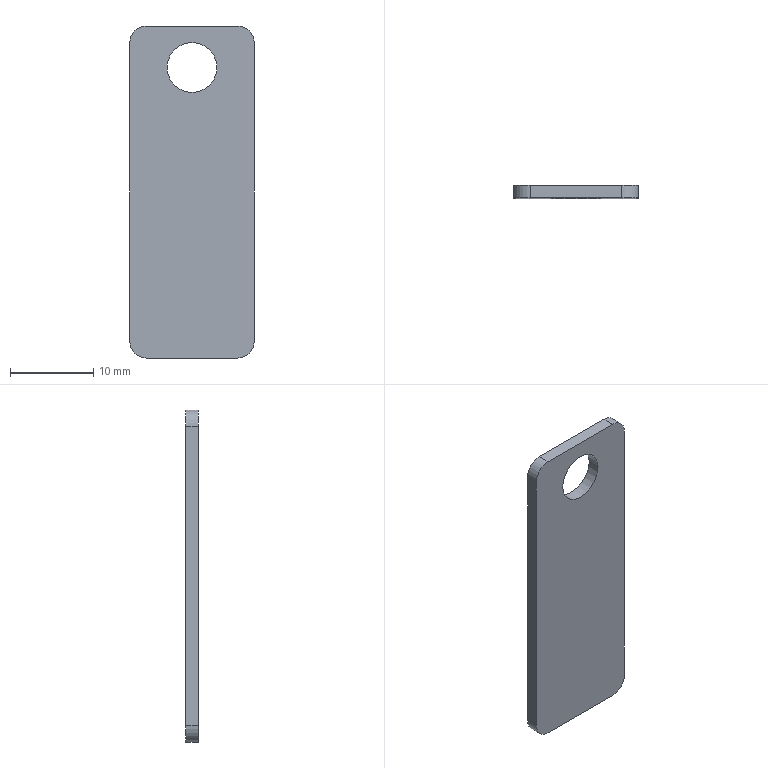Component | SolidWorks | FiberOpticBracket-1 | 1 solid | 12 faces | box 15 x 1.5 x 40 mm | volume 852 mm3 | cylinder 6 | plane 6 | commonest cylinder face diameters 4 x4 6 x2
STEP:
#1=COLOUR_RGB('',0.7922,0.8196,0.9333);
#2=FILL_AREA_STYLE_COLOUR('',#1);
#3=FILL_AREA_STYLE('',(#2));
#4=SURFACE_STYLE_FILL_AREA(#3);
#5=SURFACE_SIDE_STYLE('',(#4));
#6=SURFACE_STYLE_USAGE(.BOTH.,#5);
#7=PRESENTATION_STYLE_ASSIGNMENT((#6));
#8=CARTESIAN_POINT('',(-0.6049,-0.5041,4.668));
#9=VERTEX_POINT('',#8);
#10=CARTESIAN_POINT('',(-0.8411,-0.5041,4.668));
#11=VERTEX_POINT('',#10);
#12=CARTESIAN_POINT('',(-0.723,-0.5041,4.668));
#13=DIRECTION('',(-0.,1.,0.));
#14=DIRECTION('',(-1.,0.,0.));
#15=AXIS2_PLACEMENT_3D('',#12,#13,#14);
#16=CIRCLE('',#15,0.1181);
#17=EDGE_CURVE('',#9,#11,#16,.T.);
#18=ORIENTED_EDGE('',*,*,#17,.F.);
#19=CARTESIAN_POINT('',(-0.6049,-0.4451,4.668));
#20=VERTEX_POINT('',#19);
#21=CARTESIAN_POINT('',(-0.6049,-0.8388,4.668));
#22=DIRECTION('',(-0.,1.,0.));
#23=VECTOR('',#22,39.37);
#24=LINE('',#21,#23);
#25=EDGE_CURVE('',#9,#20,#24,.T.);
#26=ORIENTED_EDGE('',*,*,#25,.T.);
#27=CARTESIAN_POINT('',(-0.8411,-0.4451,4.668));
#28=VERTEX_POINT('',#27);
#29=CARTESIAN_POINT('',(-0.723,-0.4451,4.668));
#30=DIRECTION('',(-0.,1.,0.));
#31=DIRECTION('',(-1.,0.,0.));
#32=AXIS2_PLACEMENT_3D('',#29,#30,#31);
#33=CIRCLE('',#32,0.1181);
#34=EDGE_CURVE('',#20,#28,#33,.T.);
#35=ORIENTED_EDGE('',*,*,#34,.T.);
#36=CARTESIAN_POINT('',(-0.8411,-0.8388,4.668));
#37=DIRECTION('',(-0.,1.,0.));
#38=VECTOR('',#37,39.37);
#39=LINE('',#36,#38);
#40=EDGE_CURVE('',#11,#28,#39,.T.);
#41=ORIENTED_EDGE('',*,*,#40,.F.);
#42=EDGE_LOOP('',(#18,#26,#35,#41));
#43=FACE_OUTER_BOUND('',#42,.T.);
#44=CARTESIAN_POINT('',(-0.723,-0.8388,4.668));
#45=DIRECTION('',(-0.,1.,0.));
#46=DIRECTION('',(-1.,0.,0.));
#47=AXIS2_PLACEMENT_3D('',#44,#45,#46);
#48=CYLINDRICAL_SURFACE('',#47,0.1181);
#49=ADVANCED_FACE('',(#43),#48,.F.);
#50=CARTESIAN_POINT('',(-0.723,-0.5041,4.668));
#51=DIRECTION('',(-0.,1.,0.));
#52=DIRECTION('',(-1.,0.,0.));
#53=AXIS2_PLACEMENT_3D('',#50,#51,#52);
#54=CIRCLE('',#53,0.1181);
#55=EDGE_CURVE('',#11,#9,#54,.T.);
#56=ORIENTED_EDGE('',*,*,#55,.T.);
#57=ORIENTED_EDGE('',*,*,#17,.T.);
#58=EDGE_LOOP('',(#56,#57));
#59=FACE_BOUND('',#58,.T.);
#60=CARTESIAN_POINT('',(-0.4278,-0.5041,3.369));
#61=VERTEX_POINT('',#60);
#62=CARTESIAN_POINT('',(-0.4278,-0.5041,4.787));
#63=VERTEX_POINT('',#62);
#64=CARTESIAN_POINT('',(-0.4278,-0.5041,3.291));
#65=DIRECTION('',(-0.,-0.,1.));
#66=VECTOR('',#65,39.37);
#67=LINE('',#64,#66);
#68=EDGE_CURVE('',#61,#63,#67,.T.);
#69=ORIENTED_EDGE('',*,*,#68,.T.);
#70=CARTESIAN_POINT('',(-0.5065,-0.5041,4.865));
#71=VERTEX_POINT('',#70);
#72=CARTESIAN_POINT('',(-0.5065,-0.5041,4.787));
#73=DIRECTION('',(0.,-1.,0.));
#74=DIRECTION('',(-1.,0.,0.));
#75=AXIS2_PLACEMENT_3D('',#72,#73,#74);
#76=CIRCLE('',#75,0.07874);
#77=EDGE_CURVE('',#63,#71,#76,.T.);
#78=ORIENTED_EDGE('',*,*,#77,.T.);
#79=CARTESIAN_POINT('',(-0.9396,-0.5041,4.865));
#80=VERTEX_POINT('',#79);
#81=CARTESIAN_POINT('',(-1.018,-0.5041,4.865));
#82=DIRECTION('',(1.,0.,0.));
#83=VECTOR('',#82,39.37);
#84=LINE('',#81,#83);
#85=EDGE_CURVE('',#80,#71,#84,.T.);
#86=ORIENTED_EDGE('',*,*,#85,.F.);
#87=CARTESIAN_POINT('',(-1.018,-0.5041,4.787));
#88=VERTEX_POINT('',#87);
#89=CARTESIAN_POINT('',(-0.9396,-0.5041,4.787));
#90=DIRECTION('',(0.,-1.,0.));
#91=DIRECTION('',(-1.,0.,0.));
#92=AXIS2_PLACEMENT_3D('',#89,#90,#91);
#93=CIRCLE('',#92,0.07874);
#94=EDGE_CURVE('',#80,#88,#93,.T.);
#95=ORIENTED_EDGE('',*,*,#94,.T.);
#96=CARTESIAN_POINT('',(-1.018,-0.5041,3.369));
#97=VERTEX_POINT('',#96);
#98=CARTESIAN_POINT('',(-1.018,-0.5041,3.291));
#99=DIRECTION('',(-0.,-0.,1.));
#100=VECTOR('',#99,39.37);
#101=LINE('',#98,#100);
#102=EDGE_CURVE('',#97,#88,#101,.T.);
#103=ORIENTED_EDGE('',*,*,#102,.F.);
#104=CARTESIAN_POINT('',(-0.9396,-0.5041,3.291));
#105=VERTEX_POINT('',#104);
#106=CARTESIAN_POINT('',(-0.9396,-0.5041,3.369));
#107=DIRECTION('',(0.,-1.,0.));
#108=DIRECTION('',(-1.,0.,0.));
#109=AXIS2_PLACEMENT_3D('',#106,#107,#108);
#110=CIRCLE('',#109,0.07874);
#111=EDGE_CURVE('',#97,#105,#110,.T.);
#112=ORIENTED_EDGE('',*,*,#111,.T.);
#113=CARTESIAN_POINT('',(-0.5065,-0.5041,3.291));
#114=VERTEX_POINT('',#113);
#115=CARTESIAN_POINT('',(-1.018,-0.5041,3.291));
#116=DIRECTION('',(1.,0.,0.));
#117=VECTOR('',#116,39.37);
#118=LINE('',#115,#117);
#119=EDGE_CURVE('',#105,#114,#118,.T.);
#120=ORIENTED_EDGE('',*,*,#119,.T.);
#121=CARTESIAN_POINT('',(-0.5065,-0.5041,3.369));
#122=DIRECTION('',(0.,-1.,0.));
#123=DIRECTION('',(-1.,0.,0.));
#124=AXIS2_PLACEMENT_3D('',#121,#122,#123);
#125=CIRCLE('',#124,0.07874);
#126=EDGE_CURVE('',#114,#61,#125,.T.);
#127=ORIENTED_EDGE('',*,*,#126,.T.);
#128=EDGE_LOOP('',(#69,#78,#86,#95,#103,#112,#120,#127));
#129=FACE_OUTER_BOUND('',#128,.T.);
#130=CARTESIAN_POINT('',(-1.018,-0.5041,3.291));
#131=DIRECTION('',(-0.,1.,-0.));
#132=DIRECTION('',(-1.,-0.,-0.));
#133=AXIS2_PLACEMENT_3D('',#130,#131,#132);
#134=PLANE('',#133);
#135=ADVANCED_FACE('',(#59,#129),#134,.F.);
#136=ORIENTED_EDGE('',*,*,#85,.T.);
#137=CARTESIAN_POINT('',(-0.5065,-0.4451,4.865));
#138=VERTEX_POINT('',#137);
#139=CARTESIAN_POINT('',(-0.5065,-0.4451,4.865));
#140=DIRECTION('',(-0.,1.,0.));
#141=VECTOR('',#140,39.37);
#142=LINE('',#139,#141);
#143=EDGE_CURVE('',#71,#138,#142,.T.);
#144=ORIENTED_EDGE('',*,*,#143,.T.);
#145=CARTESIAN_POINT('',(-0.9396,-0.4451,4.865));
#146=VERTEX_POINT('',#145);
#147=CARTESIAN_POINT('',(-1.018,-0.4451,4.865));
#148=DIRECTION('',(1.,0.,0.));
#149=VECTOR('',#148,39.37);
#150=LINE('',#147,#149);
#151=EDGE_CURVE('',#146,#138,#150,.T.);
#152=ORIENTED_EDGE('',*,*,#151,.F.);
#153=CARTESIAN_POINT('',(-0.9396,-0.5041,4.865));
#154=DIRECTION('',(0.,-1.,0.));
#155=VECTOR('',#154,39.37);
#156=LINE('',#153,#155);
#157=EDGE_CURVE('',#146,#80,#156,.T.);
#158=ORIENTED_EDGE('',*,*,#157,.T.);
#159=EDGE_LOOP('',(#136,#144,#152,#158));
#160=FACE_OUTER_BOUND('',#159,.T.);
#161=CARTESIAN_POINT('',(-1.018,-0.4451,4.865));
#162=DIRECTION('',(-0.,-0.,1.));
#163=DIRECTION('',(1.,0.,0.));
#164=AXIS2_PLACEMENT_3D('',#161,#162,#163);
#165=PLANE('',#164);
#166=ADVANCED_FACE('',(#160),#165,.T.);
#167=CARTESIAN_POINT('',(-0.723,-0.4451,4.668));
#168=DIRECTION('',(-0.,1.,0.));
#169=DIRECTION('',(-1.,0.,0.));
#170=AXIS2_PLACEMENT_3D('',#167,#168,#169);
#171=CIRCLE('',#170,0.1181);
#172=EDGE_CURVE('',#28,#20,#171,.T.);
#173=ORIENTED_EDGE('',*,*,#172,.F.);
#174=ORIENTED_EDGE('',*,*,#34,.F.);
#175=EDGE_LOOP('',(#173,#174));
#176=FACE_BOUND('',#175,.T.);
#177=ORIENTED_EDGE('',*,*,#151,.T.);
#178=CARTESIAN_POINT('',(-0.4278,-0.4451,4.787));
#179=VERTEX_POINT('',#178);
#180=CARTESIAN_POINT('',(-0.5065,-0.4451,4.787));
#181=DIRECTION('',(-0.,1.,0.));
#182=DIRECTION('',(-1.,0.,0.));
#183=AXIS2_PLACEMENT_3D('',#180,#181,#182);
#184=CIRCLE('',#183,0.07874);
#185=EDGE_CURVE('',#138,#179,#184,.T.);
#186=ORIENTED_EDGE('',*,*,#185,.T.);
#187=CARTESIAN_POINT('',(-0.4278,-0.4451,3.369));
#188=VERTEX_POINT('',#187);
#189=CARTESIAN_POINT('',(-0.4278,-0.4451,3.291));
#190=DIRECTION('',(-0.,-0.,1.));
#191=VECTOR('',#190,39.37);
#192=LINE('',#189,#191);
#193=EDGE_CURVE('',#188,#179,#192,.T.);
#194=ORIENTED_EDGE('',*,*,#193,.F.);
#195=CARTESIAN_POINT('',(-0.5065,-0.4451,3.291));
#196=VERTEX_POINT('',#195);
#197=CARTESIAN_POINT('',(-0.5065,-0.4451,3.369));
#198=DIRECTION('',(-0.,1.,0.));
#199=DIRECTION('',(-1.,0.,0.));
#200=AXIS2_PLACEMENT_3D('',#197,#198,#199);
#201=CIRCLE('',#200,0.07874);
#202=EDGE_CURVE('',#188,#196,#201,.T.);
#203=ORIENTED_EDGE('',*,*,#202,.T.);
#204=CARTESIAN_POINT('',(-0.9396,-0.4451,3.291));
#205=VERTEX_POINT('',#204);
#206=CARTESIAN_POINT('',(-1.018,-0.4451,3.291));
#207=DIRECTION('',(1.,0.,0.));
#208=VECTOR('',#207,39.37);
#209=LINE('',#206,#208);
#210=EDGE_CURVE('',#205,#196,#209,.T.);
#211=ORIENTED_EDGE('',*,*,#210,.F.);
#212=CARTESIAN_POINT('',(-1.018,-0.4451,3.369));
#213=VERTEX_POINT('',#212);
#214=CARTESIAN_POINT('',(-0.9396,-0.4451,3.369));
#215=DIRECTION('',(-0.,1.,0.));
#216=DIRECTION('',(-1.,0.,0.));
#217=AXIS2_PLACEMENT_3D('',#214,#215,#216);
#218=CIRCLE('',#217,0.07874);
#219=EDGE_CURVE('',#205,#213,#218,.T.);
#220=ORIENTED_EDGE('',*,*,#219,.T.);
#221=CARTESIAN_POINT('',(-1.018,-0.4451,4.787));
#222=VERTEX_POINT('',#221);
#223=CARTESIAN_POINT('',(-1.018,-0.4451,3.291));
#224=DIRECTION('',(-0.,-0.,1.));
#225=VECTOR('',#224,39.37);
#226=LINE('',#223,#225);
#227=EDGE_CURVE('',#213,#222,#226,.T.);
#228=ORIENTED_EDGE('',*,*,#227,.T.);
#229=CARTESIAN_POINT('',(-0.9396,-0.4451,4.787));
#230=DIRECTION('',(-0.,1.,0.));
#231=DIRECTION('',(-1.,0.,0.));
#232=AXIS2_PLACEMENT_3D('',#229,#230,#231);
#233=CIRCLE('',#232,0.07874);
#234=EDGE_CURVE('',#222,#146,#233,.T.);
#235=ORIENTED_EDGE('',*,*,#234,.T.);
#236=EDGE_LOOP('',(#177,#186,#194,#203,#211,#220,#228,#235));
#237=FACE_OUTER_BOUND('',#236,.T.);
#238=CARTESIAN_POINT('',(-1.018,-0.4451,3.291));
#239=DIRECTION('',(-0.,1.,-0.));
#240=DIRECTION('',(-1.,-0.,-0.));
#241=AXIS2_PLACEMENT_3D('',#238,#239,#240);
#242=PLANE('',#241);
#243=ADVANCED_FACE('',(#176,#237),#242,.T.);
#244=ORIENTED_EDGE('',*,*,#210,.T.);
#245=CARTESIAN_POINT('',(-0.5065,-0.5041,3.291));
#246=DIRECTION('',(0.,-1.,0.));
#247=VECTOR('',#246,39.37);
#248=LINE('',#245,#247);
#249=EDGE_CURVE('',#196,#114,#248,.T.);
#250=ORIENTED_EDGE('',*,*,#249,.T.);
#251=ORIENTED_EDGE('',*,*,#119,.F.);
#252=CARTESIAN_POINT('',(-0.9396,-0.4451,3.291));
#253=DIRECTION('',(-0.,1.,0.));
#254=VECTOR('',#253,39.37);
#255=LINE('',#252,#254);
#256=EDGE_CURVE('',#105,#205,#255,.T.);
#257=ORIENTED_EDGE('',*,*,#256,.T.);
#258=EDGE_LOOP('',(#244,#250,#251,#257));
#259=FACE_OUTER_BOUND('',#258,.T.);
#260=CARTESIAN_POINT('',(-1.018,-0.5041,3.291));
#261=DIRECTION('',(0.,0.,-1.));
#262=DIRECTION('',(-1.,-0.,-0.));
#263=AXIS2_PLACEMENT_3D('',#260,#261,#262);
#264=PLANE('',#263);
#265=ADVANCED_FACE('',(#259),#264,.T.);
#266=ORIENTED_EDGE('',*,*,#102,.T.);
#267=CARTESIAN_POINT('',(-1.018,-0.4451,4.787));
#268=DIRECTION('',(-0.,1.,0.));
#269=VECTOR('',#268,39.37);
#270=LINE('',#267,#269);
#271=EDGE_CURVE('',#88,#222,#270,.T.);
#272=ORIENTED_EDGE('',*,*,#271,.T.);
#273=ORIENTED_EDGE('',*,*,#227,.F.);
#274=CARTESIAN_POINT('',(-1.018,-0.5041,3.369));
#275=DIRECTION('',(0.,-1.,0.));
#276=VECTOR('',#275,39.37);
#277=LINE('',#274,#276);
#278=EDGE_CURVE('',#213,#97,#277,.T.);
#279=ORIENTED_EDGE('',*,*,#278,.T.);
#280=EDGE_LOOP('',(#266,#272,#273,#279));
#281=FACE_OUTER_BOUND('',#280,.T.);
#282=CARTESIAN_POINT('',(-1.018,-0.4451,3.291));
#283=DIRECTION('',(1.,0.,0.));
#284=DIRECTION('',(0.,0.,-1.));
#285=AXIS2_PLACEMENT_3D('',#282,#283,#284);
#286=PLANE('',#285);
#287=ADVANCED_FACE('',(#281),#286,.F.);
#288=ORIENTED_EDGE('',*,*,#193,.T.);
#289=CARTESIAN_POINT('',(-0.4278,-0.4451,4.787));
#290=DIRECTION('',(0.,-1.,0.));
#291=VECTOR('',#290,39.37);
#292=LINE('',#289,#291);
#293=EDGE_CURVE('',#179,#63,#292,.T.);
#294=ORIENTED_EDGE('',*,*,#293,.T.);
#295=ORIENTED_EDGE('',*,*,#68,.F.);
#296=CARTESIAN_POINT('',(-0.4278,-0.4451,3.369));
#297=DIRECTION('',(-0.,1.,0.));
#298=VECTOR('',#297,39.37);
#299=LINE('',#296,#298);
#300=EDGE_CURVE('',#61,#188,#299,.T.);
#301=ORIENTED_EDGE('',*,*,#300,.T.);
#302=EDGE_LOOP('',(#288,#294,#295,#301));
#303=FACE_OUTER_BOUND('',#302,.T.);
#304=CARTESIAN_POINT('',(-0.4278,-0.4451,3.291));
#305=DIRECTION('',(1.,0.,0.));
#306=DIRECTION('',(0.,0.,-1.));
#307=AXIS2_PLACEMENT_3D('',#304,#305,#306);
#308=PLANE('',#307);
#309=ADVANCED_FACE('',(#303),#308,.T.);
#310=ORIENTED_EDGE('',*,*,#185,.F.);
#311=ORIENTED_EDGE('',*,*,#143,.F.);
#312=ORIENTED_EDGE('',*,*,#77,.F.);
#313=ORIENTED_EDGE('',*,*,#293,.F.);
#314=EDGE_LOOP('',(#310,#311,#312,#313));
#315=FACE_OUTER_BOUND('',#314,.T.);
#316=CARTESIAN_POINT('',(-0.5065,-0.4451,4.787));
#317=DIRECTION('',(0.,-1.,0.));
#318=DIRECTION('',(1.,0.,0.));
#319=AXIS2_PLACEMENT_3D('',#316,#317,#318);
#320=CYLINDRICAL_SURFACE('',#319,0.07874);
#321=ADVANCED_FACE('',(#315),#320,.T.);
#322=ORIENTED_EDGE('',*,*,#234,.F.);
#323=ORIENTED_EDGE('',*,*,#271,.F.);
#324=ORIENTED_EDGE('',*,*,#94,.F.);
#325=ORIENTED_EDGE('',*,*,#157,.F.);
#326=EDGE_LOOP('',(#322,#323,#324,#325));
#327=FACE_OUTER_BOUND('',#326,.T.);
#328=CARTESIAN_POINT('',(-0.9396,-0.4451,4.787));
#329=DIRECTION('',(-0.,1.,0.));
#330=DIRECTION('',(-1.,0.,0.));
#331=AXIS2_PLACEMENT_3D('',#328,#329,#330);
#332=CYLINDRICAL_SURFACE('',#331,0.07874);
#333=ADVANCED_FACE('',(#327),#332,.T.);
#334=ORIENTED_EDGE('',*,*,#126,.F.);
#335=ORIENTED_EDGE('',*,*,#249,.F.);
#336=ORIENTED_EDGE('',*,*,#202,.F.);
#337=ORIENTED_EDGE('',*,*,#300,.F.);
#338=EDGE_LOOP('',(#334,#335,#336,#337));
#339=FACE_OUTER_BOUND('',#338,.T.);
#340=CARTESIAN_POINT('',(-0.5065,-0.4451,3.369));
#341=DIRECTION('',(-0.,1.,0.));
#342=DIRECTION('',(-1.,0.,0.));
#343=AXIS2_PLACEMENT_3D('',#340,#341,#342);
#344=CYLINDRICAL_SURFACE('',#343,0.07874);
#345=ADVANCED_FACE('',(#339),#344,.T.);
#346=ORIENTED_EDGE('',*,*,#111,.F.);
#347=ORIENTED_EDGE('',*,*,#278,.F.);
#348=ORIENTED_EDGE('',*,*,#219,.F.);
#349=ORIENTED_EDGE('',*,*,#256,.F.);
#350=EDGE_LOOP('',(#346,#347,#348,#349));
#351=FACE_OUTER_BOUND('',#350,.T.);
#352=CARTESIAN_POINT('',(-0.9396,-0.5041,3.369));
#353=DIRECTION('',(0.,-1.,0.));
#354=DIRECTION('',(1.,0.,0.));
#355=AXIS2_PLACEMENT_3D('',#352,#353,#354);
#356=CYLINDRICAL_SURFACE('',#355,0.07874);
#357=ADVANCED_FACE('',(#351),#356,.T.);
#358=ORIENTED_EDGE('',*,*,#25,.F.);
#359=ORIENTED_EDGE('',*,*,#55,.F.);
#360=ORIENTED_EDGE('',*,*,#40,.T.);
#361=ORIENTED_EDGE('',*,*,#172,.T.);
#362=EDGE_LOOP('',(#358,#359,#360,#361));
#363=FACE_OUTER_BOUND('',#362,.T.);
#364=CARTESIAN_POINT('',(-0.723,-0.8388,4.668));
#365=DIRECTION('',(-0.,1.,0.));
#366=DIRECTION('',(-1.,0.,0.));
#367=AXIS2_PLACEMENT_3D('',#364,#365,#366);
#368=CYLINDRICAL_SURFACE('',#367,0.1181);
#369=ADVANCED_FACE('',(#363),#368,.F.);
#370=CLOSED_SHELL('',(#49,#135,#166,#243,#265,#287,#309,#321,#333,#345,#357,#369));
#371=MANIFOLD_SOLID_BREP('',#370);
#372=STYLED_ITEM('',(#7),#371);
#373=(LENGTH_UNIT()NAMED_UNIT(*)SI_UNIT($,.METRE.));
#374=LENGTH_MEASURE_WITH_UNIT(LENGTH_MEASURE(0.0254),#373);
#375=DIMENSIONAL_EXPONENTS(1.,0.,0.,0.,0.,0.,0.);
#376=(CONVERSION_BASED_UNIT('',#374)LENGTH_UNIT()NAMED_UNIT(#375));
#377=UNCERTAINTY_MEASURE_WITH_UNIT(LENGTH_MEASURE(0.00001),#376,'','');
#378=(NAMED_UNIT(*)PLANE_ANGLE_UNIT()SI_UNIT($,.RADIAN.));
#379=(NAMED_UNIT(*)SI_UNIT($,.STERADIAN.)SOLID_ANGLE_UNIT());
#380=(GEOMETRIC_REPRESENTATION_CONTEXT(3)GLOBAL_UNCERTAINTY_ASSIGNED_CONTEXT((#377))GLOBAL_UNIT_ASSIGNED_CONTEXT((#376,#378,#379))REPRESENTATION_CONTEXT('',''));
#381=MECHANICAL_DESIGN_GEOMETRIC_PRESENTATION_REPRESENTATION('',(#372),#380);
#382=PRESENTATION_LAYER_ASSIGNMENT('','',(#372));
#383=CARTESIAN_POINT('',(0.,0.,0.));
#384=DIRECTION('',(0.,0.,1.));
#385=DIRECTION('',(1.,0.,0.));
#386=AXIS2_PLACEMENT_3D('',#383,#384,#385);
#387=(LENGTH_UNIT()NAMED_UNIT(*)SI_UNIT($,.METRE.));
#388=LENGTH_MEASURE_WITH_UNIT(LENGTH_MEASURE(0.0254),#387);
#389=DIMENSIONAL_EXPONENTS(1.,0.,0.,0.,0.,0.,0.);
#390=(CONVERSION_BASED_UNIT('',#388)LENGTH_UNIT()NAMED_UNIT(#389));
#391=UNCERTAINTY_MEASURE_WITH_UNIT(LENGTH_MEASURE(0.00001),#390,'','');
#392=(NAMED_UNIT(*)PLANE_ANGLE_UNIT()SI_UNIT($,.RADIAN.));
#393=(NAMED_UNIT(*)SI_UNIT($,.STERADIAN.)SOLID_ANGLE_UNIT());
#394=(GEOMETRIC_REPRESENTATION_CONTEXT(3)GLOBAL_UNCERTAINTY_ASSIGNED_CONTEXT((#391))GLOBAL_UNIT_ASSIGNED_CONTEXT((#390,#392,#393))REPRESENTATION_CONTEXT('',''));
#395=ADVANCED_BREP_SHAPE_REPRESENTATION('',(#371,#386),#394);